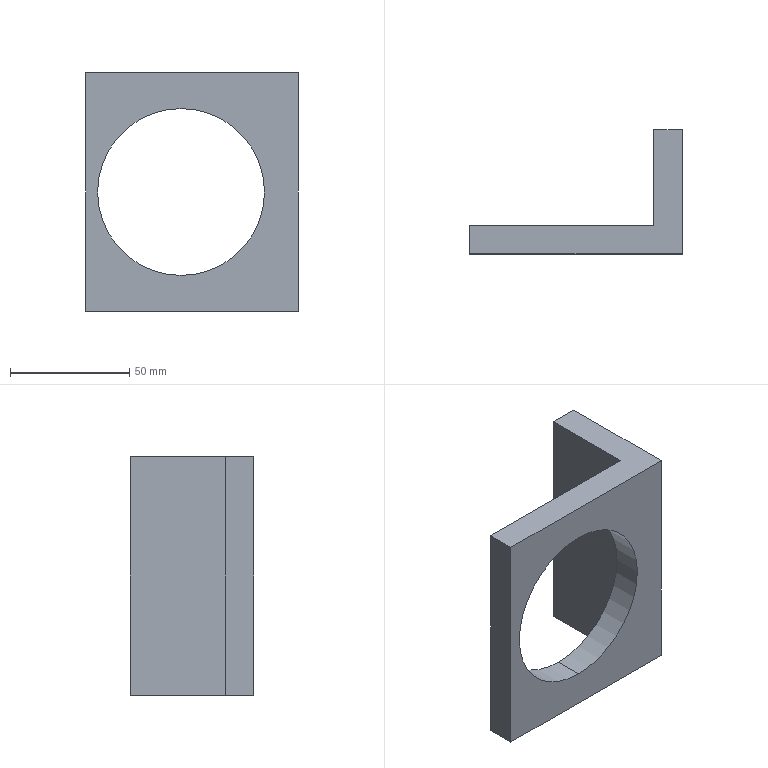Component | SolidWorks | RotatingMotorFixingPlate-1 | 1 solid | 10 faces | box 89.2 x 52 x 100 mm | volume 108859 mm3 | plane 8 | cylinder 2 | commonest cylinder face diameters 70 x2 | material Plain Carbon Steel
build123d program:
from build123d import *

# Parameters (mm, degrees)
SKETCH1_W           = 100
SKETCH1_H           = 89.2
BOSS_EXTRUDE1_DEPTH = 12
SKETCH2_W           = 100
SKETCH2_H           = 12
BOSS_EXTRUDE2_DEPTH = 40
SKETCH3_R           = 35
CUT_EXTRUDE1_DEPTH  = 79.033


with BuildPart() as part:
    # Sketch1 → Boss-Extrude1 (new body)
    with BuildSketch(Plane.XY):
        Rectangle(SKETCH1_W, SKETCH1_H)
    extrude(amount=BOSS_EXTRUDE1_DEPTH)

    # Sketch2 → Boss-Extrude2 (add)
    with BuildSketch(Plane.XY.offset(12)):
        with Locations((0, -38.6)):
            Rectangle(SKETCH2_W, SKETCH2_H)
    extrude(amount=BOSS_EXTRUDE2_DEPTH)

    # Sketch3 → Cut-Extrude1 (cut, through all)
    with BuildSketch(Plane.XY.offset(12)):
        with Locations((0, 4.6)):
            Circle(SKETCH3_R)
    extrude(amount=-CUT_EXTRUDE1_DEPTH, mode=Mode.SUBTRACT)


solid = part.part

# Placed as in the assembly
solid = solid.moved(Location((-860.285, -524.907, 1035.102), (-90, 0, 90)))
STEP:
#1=COLOUR_RGB('',0.7922,0.8196,0.9333);
#2=FILL_AREA_STYLE_COLOUR('',#1);
#3=FILL_AREA_STYLE('',(#2));
#4=SURFACE_STYLE_FILL_AREA(#3);
#5=SURFACE_SIDE_STYLE('',(#4));
#6=SURFACE_STYLE_USAGE(.BOTH.,#5);
#7=PRESENTATION_STYLE_ASSIGNMENT((#6));
#8=CARTESIAN_POINT('',(-34.051,-20.666,42.13));
#9=VERTEX_POINT('',#8);
#10=CARTESIAN_POINT('',(-34.051,-20.666,39.374));
#11=VERTEX_POINT('',#10);
#12=CARTESIAN_POINT('',(-34.051,-20.666,40.752));
#13=DIRECTION('',(0.,1.,0.));
#14=DIRECTION('',(0.,0.,-1.));
#15=AXIS2_PLACEMENT_3D('',#12,#13,#14);
#16=CIRCLE('',#15,1.378);
#17=EDGE_CURVE('',#9,#11,#16,.T.);
#18=ORIENTED_EDGE('',*,*,#17,.F.);
#19=CARTESIAN_POINT('',(-34.051,-20.193,42.13));
#20=VERTEX_POINT('',#19);
#21=CARTESIAN_POINT('',(-34.051,-20.666,42.13));
#22=DIRECTION('',(0.,1.,0.));
#23=VECTOR('',#22,39.37);
#24=LINE('',#21,#23);
#25=EDGE_CURVE('',#9,#20,#24,.T.);
#26=ORIENTED_EDGE('',*,*,#25,.T.);
#27=CARTESIAN_POINT('',(-34.051,-20.193,39.374));
#28=VERTEX_POINT('',#27);
#29=CARTESIAN_POINT('',(-34.051,-20.193,40.752));
#30=DIRECTION('',(0.,1.,0.));
#31=DIRECTION('',(0.,0.,-1.));
#32=AXIS2_PLACEMENT_3D('',#29,#30,#31);
#33=CIRCLE('',#32,1.378);
#34=EDGE_CURVE('',#20,#28,#33,.T.);
#35=ORIENTED_EDGE('',*,*,#34,.T.);
#36=CARTESIAN_POINT('',(-34.051,-20.666,39.374));
#37=DIRECTION('',(0.,1.,0.));
#38=VECTOR('',#37,39.37);
#39=LINE('',#36,#38);
#40=EDGE_CURVE('',#11,#28,#39,.T.);
#41=ORIENTED_EDGE('',*,*,#40,.F.);
#42=EDGE_LOOP('',(#18,#26,#35,#41));
#43=FACE_OUTER_BOUND('',#42,.T.);
#44=CARTESIAN_POINT('',(-34.051,-20.666,40.752));
#45=DIRECTION('',(0.,1.,0.));
#46=DIRECTION('',(0.,0.,-1.));
#47=AXIS2_PLACEMENT_3D('',#44,#45,#46);
#48=CYLINDRICAL_SURFACE('',#47,1.378);
#49=ADVANCED_FACE('',(#43),#48,.F.);
#50=CARTESIAN_POINT('',(-35.625,-20.666,42.721));
#51=VERTEX_POINT('',#50);
#52=CARTESIAN_POINT('',(-32.114,-20.666,42.721));
#53=VERTEX_POINT('',#52);
#54=CARTESIAN_POINT('',(-32.114,-20.666,42.721));
#55=DIRECTION('',(1.,-0.,-0.));
#56=VECTOR('',#55,39.37);
#57=LINE('',#54,#56);
#58=EDGE_CURVE('',#51,#53,#57,.T.);
#59=ORIENTED_EDGE('',*,*,#58,.T.);
#60=CARTESIAN_POINT('',(-32.114,-18.618,42.721));
#61=VERTEX_POINT('',#60);
#62=CARTESIAN_POINT('',(-32.114,-20.193,42.721));
#63=DIRECTION('',(-0.,-1.,-0.));
#64=VECTOR('',#63,39.37);
#65=LINE('',#62,#64);
#66=EDGE_CURVE('',#61,#53,#65,.T.);
#67=ORIENTED_EDGE('',*,*,#66,.F.);
#68=CARTESIAN_POINT('',(-32.586,-18.618,42.721));
#69=VERTEX_POINT('',#68);
#70=CARTESIAN_POINT('',(-32.114,-18.618,42.721));
#71=DIRECTION('',(1.,-0.,-0.));
#72=VECTOR('',#71,39.37);
#73=LINE('',#70,#72);
#74=EDGE_CURVE('',#69,#61,#73,.T.);
#75=ORIENTED_EDGE('',*,*,#74,.F.);
#76=CARTESIAN_POINT('',(-32.586,-20.193,42.721));
#77=VERTEX_POINT('',#76);
#78=CARTESIAN_POINT('',(-32.586,-18.618,42.721));
#79=DIRECTION('',(-0.,-1.,-0.));
#80=VECTOR('',#79,39.37);
#81=LINE('',#78,#80);
#82=EDGE_CURVE('',#69,#77,#81,.T.);
#83=ORIENTED_EDGE('',*,*,#82,.T.);
#84=CARTESIAN_POINT('',(-35.625,-20.193,42.721));
#85=VERTEX_POINT('',#84);
#86=CARTESIAN_POINT('',(-32.114,-20.193,42.721));
#87=DIRECTION('',(1.,-0.,-0.));
#88=VECTOR('',#87,39.37);
#89=LINE('',#86,#88);
#90=EDGE_CURVE('',#85,#77,#89,.T.);
#91=ORIENTED_EDGE('',*,*,#90,.F.);
#92=CARTESIAN_POINT('',(-35.625,-20.193,42.721));
#93=DIRECTION('',(-0.,-1.,-0.));
#94=VECTOR('',#93,39.37);
#95=LINE('',#92,#94);
#96=EDGE_CURVE('',#85,#51,#95,.T.);
#97=ORIENTED_EDGE('',*,*,#96,.T.);
#98=EDGE_LOOP('',(#59,#67,#75,#83,#91,#97));
#99=FACE_OUTER_BOUND('',#98,.T.);
#100=CARTESIAN_POINT('',(-32.114,-20.193,42.721));
#101=DIRECTION('',(-0.,0.,-1.));
#102=DIRECTION('',(-0.,-1.,-0.));
#103=AXIS2_PLACEMENT_3D('',#100,#101,#102);
#104=PLANE('',#103);
#105=ADVANCED_FACE('',(#99),#104,.F.);
#106=CARTESIAN_POINT('',(-32.114,-20.666,38.784));
#107=VERTEX_POINT('',#106);
#108=CARTESIAN_POINT('',(-32.114,-20.666,38.784));
#109=DIRECTION('',(-0.,0.,-1.));
#110=VECTOR('',#109,39.37);
#111=LINE('',#108,#110);
#112=EDGE_CURVE('',#53,#107,#111,.T.);
#113=ORIENTED_EDGE('',*,*,#112,.T.);
#114=CARTESIAN_POINT('',(-32.114,-18.618,38.784));
#115=VERTEX_POINT('',#114);
#116=CARTESIAN_POINT('',(-32.114,-20.193,38.784));
#117=DIRECTION('',(-0.,-1.,-0.));
#118=VECTOR('',#117,39.37);
#119=LINE('',#116,#118);
#120=EDGE_CURVE('',#115,#107,#119,.T.);
#121=ORIENTED_EDGE('',*,*,#120,.F.);
#122=CARTESIAN_POINT('',(-32.114,-18.618,42.721));
#123=DIRECTION('',(-0.,0.,-1.));
#124=VECTOR('',#123,39.37);
#125=LINE('',#122,#124);
#126=EDGE_CURVE('',#61,#115,#125,.T.);
#127=ORIENTED_EDGE('',*,*,#126,.F.);
#128=ORIENTED_EDGE('',*,*,#66,.T.);
#129=EDGE_LOOP('',(#113,#121,#127,#128));
#130=FACE_OUTER_BOUND('',#129,.T.);
#131=CARTESIAN_POINT('',(-32.114,-20.193,38.784));
#132=DIRECTION('',(-1.,0.,0.));
#133=DIRECTION('',(0.,-0.,1.));
#134=AXIS2_PLACEMENT_3D('',#131,#132,#133);
#135=PLANE('',#134);
#136=ADVANCED_FACE('',(#130),#135,.F.);
#137=CARTESIAN_POINT('',(-35.625,-20.666,38.784));
#138=VERTEX_POINT('',#137);
#139=CARTESIAN_POINT('',(-32.114,-20.666,38.784));
#140=DIRECTION('',(-1.,0.,0.));
#141=VECTOR('',#140,39.37);
#142=LINE('',#139,#141);
#143=EDGE_CURVE('',#107,#138,#142,.T.);
#144=ORIENTED_EDGE('',*,*,#143,.T.);
#145=CARTESIAN_POINT('',(-35.625,-20.193,38.784));
#146=VERTEX_POINT('',#145);
#147=CARTESIAN_POINT('',(-35.625,-20.193,38.784));
#148=DIRECTION('',(-0.,-1.,-0.));
#149=VECTOR('',#148,39.37);
#150=LINE('',#147,#149);
#151=EDGE_CURVE('',#146,#138,#150,.T.);
#152=ORIENTED_EDGE('',*,*,#151,.F.);
#153=CARTESIAN_POINT('',(-32.586,-20.193,38.784));
#154=VERTEX_POINT('',#153);
#155=CARTESIAN_POINT('',(-32.114,-20.193,38.784));
#156=DIRECTION('',(-1.,0.,0.));
#157=VECTOR('',#156,39.37);
#158=LINE('',#155,#157);
#159=EDGE_CURVE('',#154,#146,#158,.T.);
#160=ORIENTED_EDGE('',*,*,#159,.F.);
#161=CARTESIAN_POINT('',(-32.586,-18.618,38.784));
#162=VERTEX_POINT('',#161);
#163=CARTESIAN_POINT('',(-32.586,-18.618,38.784));
#164=DIRECTION('',(-0.,-1.,-0.));
#165=VECTOR('',#164,39.37);
#166=LINE('',#163,#165);
#167=EDGE_CURVE('',#162,#154,#166,.T.);
#168=ORIENTED_EDGE('',*,*,#167,.F.);
#169=CARTESIAN_POINT('',(-32.114,-18.618,38.784));
#170=DIRECTION('',(-1.,0.,0.));
#171=VECTOR('',#170,39.37);
#172=LINE('',#169,#171);
#173=EDGE_CURVE('',#115,#162,#172,.T.);
#174=ORIENTED_EDGE('',*,*,#173,.F.);
#175=ORIENTED_EDGE('',*,*,#120,.T.);
#176=EDGE_LOOP('',(#144,#152,#160,#168,#174,#175));
#177=FACE_OUTER_BOUND('',#176,.T.);
#178=CARTESIAN_POINT('',(-32.114,-20.193,38.784));
#179=DIRECTION('',(0.,-0.,1.));
#180=DIRECTION('',(0.,1.,0.));
#181=AXIS2_PLACEMENT_3D('',#178,#179,#180);
#182=PLANE('',#181);
#183=ADVANCED_FACE('',(#177),#182,.F.);
#184=CARTESIAN_POINT('',(-35.625,-20.666,38.784));
#185=DIRECTION('',(0.,-0.,1.));
#186=VECTOR('',#185,39.37);
#187=LINE('',#184,#186);
#188=EDGE_CURVE('',#138,#51,#187,.T.);
#189=ORIENTED_EDGE('',*,*,#188,.T.);
#190=ORIENTED_EDGE('',*,*,#96,.F.);
#191=CARTESIAN_POINT('',(-35.625,-20.193,38.784));
#192=DIRECTION('',(0.,-0.,1.));
#193=VECTOR('',#192,39.37);
#194=LINE('',#191,#193);
#195=EDGE_CURVE('',#146,#85,#194,.T.);
#196=ORIENTED_EDGE('',*,*,#195,.F.);
#197=ORIENTED_EDGE('',*,*,#151,.T.);
#198=EDGE_LOOP('',(#189,#190,#196,#197));
#199=FACE_OUTER_BOUND('',#198,.T.);
#200=CARTESIAN_POINT('',(-35.625,-20.193,38.784));
#201=DIRECTION('',(1.,-0.,-0.));
#202=DIRECTION('',(-0.,0.,-1.));
#203=AXIS2_PLACEMENT_3D('',#200,#201,#202);
#204=PLANE('',#203);
#205=ADVANCED_FACE('',(#199),#204,.F.);
#206=CARTESIAN_POINT('',(-34.051,-20.193,40.752));
#207=DIRECTION('',(0.,1.,0.));
#208=DIRECTION('',(0.,0.,-1.));
#209=AXIS2_PLACEMENT_3D('',#206,#207,#208);
#210=CIRCLE('',#209,1.378);
#211=EDGE_CURVE('',#28,#20,#210,.T.);
#212=ORIENTED_EDGE('',*,*,#211,.F.);
#213=ORIENTED_EDGE('',*,*,#34,.F.);
#214=EDGE_LOOP('',(#212,#213));
#215=FACE_BOUND('',#214,.T.);
#216=CARTESIAN_POINT('',(-32.586,-20.193,42.721));
#217=DIRECTION('',(0.,-0.,1.));
#218=VECTOR('',#217,39.37);
#219=LINE('',#216,#218);
#220=EDGE_CURVE('',#154,#77,#219,.T.);
#221=ORIENTED_EDGE('',*,*,#220,.F.);
#222=ORIENTED_EDGE('',*,*,#159,.T.);
#223=ORIENTED_EDGE('',*,*,#195,.T.);
#224=ORIENTED_EDGE('',*,*,#90,.T.);
#225=EDGE_LOOP('',(#221,#222,#223,#224));
#226=FACE_OUTER_BOUND('',#225,.T.);
#227=CARTESIAN_POINT('',(-33.869,-20.193,40.752));
#228=DIRECTION('',(0.,1.,0.));
#229=DIRECTION('',(-0.,0.,-1.));
#230=AXIS2_PLACEMENT_3D('',#227,#228,#229);
#231=PLANE('',#230);
#232=ADVANCED_FACE('',(#215,#226),#231,.T.);
#233=CARTESIAN_POINT('',(-34.051,-20.666,40.752));
#234=DIRECTION('',(0.,1.,0.));
#235=DIRECTION('',(0.,0.,-1.));
#236=AXIS2_PLACEMENT_3D('',#233,#234,#235);
#237=CIRCLE('',#236,1.378);
#238=EDGE_CURVE('',#11,#9,#237,.T.);
#239=ORIENTED_EDGE('',*,*,#238,.T.);
#240=ORIENTED_EDGE('',*,*,#17,.T.);
#241=EDGE_LOOP('',(#239,#240));
#242=FACE_BOUND('',#241,.T.);
#243=ORIENTED_EDGE('',*,*,#58,.F.);
#244=ORIENTED_EDGE('',*,*,#188,.F.);
#245=ORIENTED_EDGE('',*,*,#143,.F.);
#246=ORIENTED_EDGE('',*,*,#112,.F.);
#247=EDGE_LOOP('',(#243,#244,#245,#246));
#248=FACE_OUTER_BOUND('',#247,.T.);
#249=CARTESIAN_POINT('',(-33.869,-20.666,40.752));
#250=DIRECTION('',(0.,1.,0.));
#251=DIRECTION('',(-0.,0.,-1.));
#252=AXIS2_PLACEMENT_3D('',#249,#250,#251);
#253=PLANE('',#252);
#254=ADVANCED_FACE('',(#242,#248),#253,.F.);
#255=ORIENTED_EDGE('',*,*,#220,.T.);
#256=ORIENTED_EDGE('',*,*,#82,.F.);
#257=CARTESIAN_POINT('',(-32.586,-18.618,42.721));
#258=DIRECTION('',(0.,-0.,1.));
#259=VECTOR('',#258,39.37);
#260=LINE('',#257,#259);
#261=EDGE_CURVE('',#162,#69,#260,.T.);
#262=ORIENTED_EDGE('',*,*,#261,.F.);
#263=ORIENTED_EDGE('',*,*,#167,.T.);
#264=EDGE_LOOP('',(#255,#256,#262,#263));
#265=FACE_OUTER_BOUND('',#264,.T.);
#266=CARTESIAN_POINT('',(-32.586,-18.618,42.721));
#267=DIRECTION('',(1.,-0.,-0.));
#268=DIRECTION('',(-0.,-1.,-0.));
#269=AXIS2_PLACEMENT_3D('',#266,#267,#268);
#270=PLANE('',#269);
#271=ADVANCED_FACE('',(#265),#270,.F.);
#272=ORIENTED_EDGE('',*,*,#74,.T.);
#273=ORIENTED_EDGE('',*,*,#126,.T.);
#274=ORIENTED_EDGE('',*,*,#173,.T.);
#275=ORIENTED_EDGE('',*,*,#261,.T.);
#276=EDGE_LOOP('',(#272,#273,#274,#275));
#277=FACE_OUTER_BOUND('',#276,.T.);
#278=CARTESIAN_POINT('',(-33.869,-18.618,40.752));
#279=DIRECTION('',(-0.,-1.,-0.));
#280=DIRECTION('',(0.,-0.,1.));
#281=AXIS2_PLACEMENT_3D('',#278,#279,#280);
#282=PLANE('',#281);
#283=ADVANCED_FACE('',(#277),#282,.F.);
#284=ORIENTED_EDGE('',*,*,#25,.F.);
#285=ORIENTED_EDGE('',*,*,#238,.F.);
#286=ORIENTED_EDGE('',*,*,#40,.T.);
#287=ORIENTED_EDGE('',*,*,#211,.T.);
#288=EDGE_LOOP('',(#284,#285,#286,#287));
#289=FACE_OUTER_BOUND('',#288,.T.);
#290=CARTESIAN_POINT('',(-34.051,-20.666,40.752));
#291=DIRECTION('',(0.,1.,0.));
#292=DIRECTION('',(0.,0.,-1.));
#293=AXIS2_PLACEMENT_3D('',#290,#291,#292);
#294=CYLINDRICAL_SURFACE('',#293,1.378);
#295=ADVANCED_FACE('',(#289),#294,.F.);
#296=CLOSED_SHELL('',(#49,#105,#136,#183,#205,#232,#254,#271,#283,#295));
#297=MANIFOLD_SOLID_BREP('',#296);
#298=STYLED_ITEM('',(#7),#297);
#299=(LENGTH_UNIT()NAMED_UNIT(*)SI_UNIT($,.METRE.));
#300=LENGTH_MEASURE_WITH_UNIT(LENGTH_MEASURE(0.0254),#299);
#301=DIMENSIONAL_EXPONENTS(1.,0.,0.,0.,0.,0.,0.);
#302=(CONVERSION_BASED_UNIT('',#300)LENGTH_UNIT()NAMED_UNIT(#301));
#303=UNCERTAINTY_MEASURE_WITH_UNIT(LENGTH_MEASURE(0.00001),#302,'','');
#304=(NAMED_UNIT(*)PLANE_ANGLE_UNIT()SI_UNIT($,.RADIAN.));
#305=(NAMED_UNIT(*)SI_UNIT($,.STERADIAN.)SOLID_ANGLE_UNIT());
#306=(GEOMETRIC_REPRESENTATION_CONTEXT(3)GLOBAL_UNCERTAINTY_ASSIGNED_CONTEXT((#303))GLOBAL_UNIT_ASSIGNED_CONTEXT((#302,#304,#305))REPRESENTATION_CONTEXT('',''));
#307=MECHANICAL_DESIGN_GEOMETRIC_PRESENTATION_REPRESENTATION('',(#298),#306);
#308=PRESENTATION_LAYER_ASSIGNMENT('','',(#298));
#309=CARTESIAN_POINT('',(0.,0.,0.));
#310=DIRECTION('',(0.,0.,1.));
#311=DIRECTION('',(1.,0.,0.));
#312=AXIS2_PLACEMENT_3D('',#309,#310,#311);
#313=(LENGTH_UNIT()NAMED_UNIT(*)SI_UNIT($,.METRE.));
#314=LENGTH_MEASURE_WITH_UNIT(LENGTH_MEASURE(0.0254),#313);
#315=DIMENSIONAL_EXPONENTS(1.,0.,0.,0.,0.,0.,0.);
#316=(CONVERSION_BASED_UNIT('',#314)LENGTH_UNIT()NAMED_UNIT(#315));
#317=UNCERTAINTY_MEASURE_WITH_UNIT(LENGTH_MEASURE(0.00001),#316,'','');
#318=(NAMED_UNIT(*)PLANE_ANGLE_UNIT()SI_UNIT($,.RADIAN.));
#319=(NAMED_UNIT(*)SI_UNIT($,.STERADIAN.)SOLID_ANGLE_UNIT());
#320=(GEOMETRIC_REPRESENTATION_CONTEXT(3)GLOBAL_UNCERTAINTY_ASSIGNED_CONTEXT((#317))GLOBAL_UNIT_ASSIGNED_CONTEXT((#316,#318,#319))REPRESENTATION_CONTEXT('',''));
#321=ADVANCED_BREP_SHAPE_REPRESENTATION('',(#297,#312),#320);